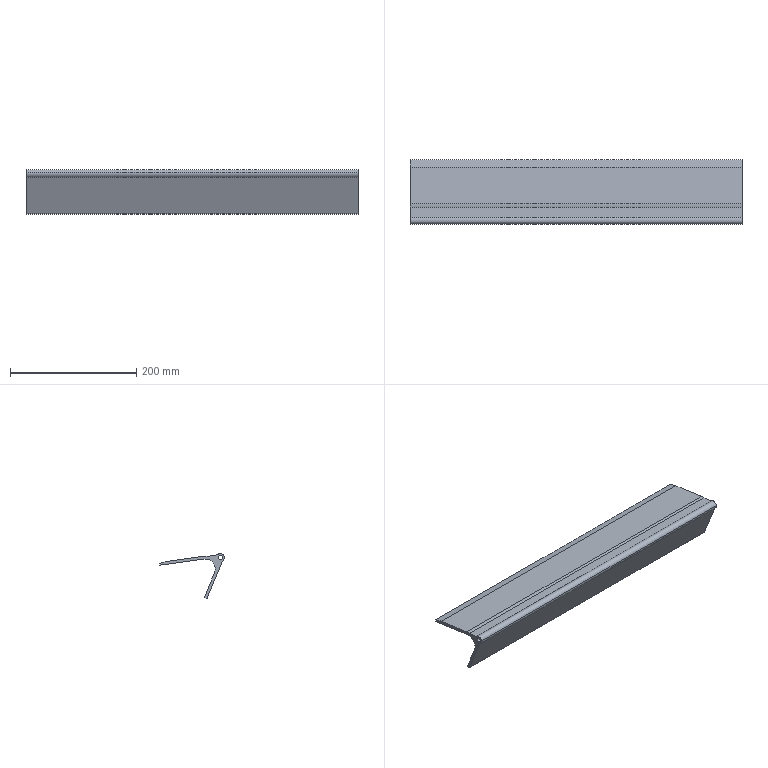Component | SolidWorks | DNR-71M20100BBEF2xx-A_501077-1 | 1 solid | 18 faces | box 525.45 x 102.87 x 71.23 mm | volume 480800 mm3 | plane 10 | cylinder 8 | commonest cylinder face diameters 12.7 x2 6.528 x2 31.496 x2 2.54 x1 40.64 x1
STEP:
#1=COLOUR_RGB('',0.7922,0.8196,0.9333);
#2=FILL_AREA_STYLE_COLOUR('',#1);
#3=FILL_AREA_STYLE('',(#2));
#4=SURFACE_STYLE_FILL_AREA(#3);
#5=SURFACE_SIDE_STYLE('',(#4));
#6=SURFACE_STYLE_USAGE(.BOTH.,#5);
#7=PRESENTATION_STYLE_ASSIGNMENT((#6));
#8=CARTESIAN_POINT('',(-10.343,-7.315,8.301));
#9=VERTEX_POINT('',#8);
#10=CARTESIAN_POINT('',(-10.343,-6.88,8.433));
#11=VERTEX_POINT('',#10);
#12=CARTESIAN_POINT('',(-10.343,-7.067,8.267));
#13=DIRECTION('',(-1.,-0.,0.));
#14=DIRECTION('',(0.,-0.9906,0.1369));
#15=AXIS2_PLACEMENT_3D('',#12,#13,#14);
#16=CIRCLE('',#15,0.25);
#17=EDGE_CURVE('',#9,#11,#16,.T.);
#18=ORIENTED_EDGE('',*,*,#17,.F.);
#19=CARTESIAN_POINT('',(10.343,-7.315,8.301));
#20=VERTEX_POINT('',#19);
#21=CARTESIAN_POINT('',(-11.051,-7.315,8.301));
#22=DIRECTION('',(1.,0.,-0.));
#23=VECTOR('',#22,39.37);
#24=LINE('',#21,#23);
#25=EDGE_CURVE('',#9,#20,#24,.T.);
#26=ORIENTED_EDGE('',*,*,#25,.T.);
#27=CARTESIAN_POINT('',(10.343,-6.88,8.433));
#28=VERTEX_POINT('',#27);
#29=CARTESIAN_POINT('',(10.343,-7.067,8.267));
#30=DIRECTION('',(1.,0.,-0.));
#31=DIRECTION('',(0.,-0.9906,0.1369));
#32=AXIS2_PLACEMENT_3D('',#29,#30,#31);
#33=CIRCLE('',#32,0.25);
#34=EDGE_CURVE('',#28,#20,#33,.T.);
#35=ORIENTED_EDGE('',*,*,#34,.F.);
#36=CARTESIAN_POINT('',(-11.051,-6.88,8.433));
#37=DIRECTION('',(-1.,-0.,0.));
#38=VECTOR('',#37,39.37);
#39=LINE('',#36,#38);
#40=EDGE_CURVE('',#28,#11,#39,.T.);
#41=ORIENTED_EDGE('',*,*,#40,.T.);
#42=EDGE_LOOP('',(#18,#26,#35,#41));
#43=FACE_OUTER_BOUND('',#42,.T.);
#44=CARTESIAN_POINT('',(-11.051,-7.067,8.267));
#45=DIRECTION('',(1.,0.,-0.));
#46=DIRECTION('',(0.,-0.9906,0.1369));
#47=AXIS2_PLACEMENT_3D('',#44,#45,#46);
#48=CYLINDRICAL_SURFACE('',#47,0.25);
#49=ADVANCED_FACE('',(#43),#48,.T.);
#50=CARTESIAN_POINT('',(-10.343,-7.194,8.285));
#51=VERTEX_POINT('',#50);
#52=CARTESIAN_POINT('',(-10.343,-6.94,8.25));
#53=VERTEX_POINT('',#52);
#54=CARTESIAN_POINT('',(-10.343,-7.067,8.267));
#55=DIRECTION('',(-1.,-0.,0.));
#56=DIRECTION('',(0.,-0.9906,0.1369));
#57=AXIS2_PLACEMENT_3D('',#54,#55,#56);
#58=CIRCLE('',#57,0.1285);
#59=EDGE_CURVE('',#51,#53,#58,.T.);
#60=ORIENTED_EDGE('',*,*,#59,.T.);
#61=CARTESIAN_POINT('',(10.343,-6.94,8.25));
#62=VERTEX_POINT('',#61);
#63=CARTESIAN_POINT('',(-11.891,-6.94,8.25));
#64=DIRECTION('',(1.,0.,-0.));
#65=VECTOR('',#64,39.37);
#66=LINE('',#63,#65);
#67=EDGE_CURVE('',#53,#62,#66,.T.);
#68=ORIENTED_EDGE('',*,*,#67,.T.);
#69=CARTESIAN_POINT('',(10.343,-7.194,8.285));
#70=VERTEX_POINT('',#69);
#71=CARTESIAN_POINT('',(10.343,-7.067,8.267));
#72=DIRECTION('',(1.,0.,-0.));
#73=DIRECTION('',(0.,-0.9906,0.1369));
#74=AXIS2_PLACEMENT_3D('',#71,#72,#73);
#75=CIRCLE('',#74,0.1285);
#76=EDGE_CURVE('',#62,#70,#75,.T.);
#77=ORIENTED_EDGE('',*,*,#76,.T.);
#78=CARTESIAN_POINT('',(-11.891,-7.194,8.285));
#79=DIRECTION('',(1.,0.,-0.));
#80=VECTOR('',#79,39.37);
#81=LINE('',#78,#80);
#82=EDGE_CURVE('',#51,#70,#81,.T.);
#83=ORIENTED_EDGE('',*,*,#82,.F.);
#84=EDGE_LOOP('',(#60,#68,#77,#83));
#85=FACE_OUTER_BOUND('',#84,.T.);
#86=CARTESIAN_POINT('',(-11.891,-7.067,8.267));
#87=DIRECTION('',(1.,0.,-0.));
#88=DIRECTION('',(0.,-0.9906,0.1369));
#89=AXIS2_PLACEMENT_3D('',#86,#87,#88);
#90=CYLINDRICAL_SURFACE('',#89,0.1285);
#91=ADVANCED_FACE('',(#85),#90,.F.);
#92=CARTESIAN_POINT('',(-10.343,-6.691,7.317));
#93=VERTEX_POINT('',#92);
#94=CARTESIAN_POINT('',(-10.343,-6.731,7.635));
#95=VERTEX_POINT('',#94);
#96=CARTESIAN_POINT('',(-10.343,-6.117,7.55));
#97=DIRECTION('',(-1.,-0.,0.));
#98=DIRECTION('',(0.,-0.9906,0.1369));
#99=AXIS2_PLACEMENT_3D('',#96,#97,#98);
#100=CIRCLE('',#99,0.62);
#101=EDGE_CURVE('',#93,#95,#100,.T.);
#102=ORIENTED_EDGE('',*,*,#101,.T.);
#103=CARTESIAN_POINT('',(10.343,-6.731,7.635));
#104=VERTEX_POINT('',#103);
#105=CARTESIAN_POINT('',(-10.343,-6.731,7.635));
#106=DIRECTION('',(1.,0.,-0.));
#107=VECTOR('',#106,39.37);
#108=LINE('',#105,#107);
#109=EDGE_CURVE('',#95,#104,#108,.T.);
#110=ORIENTED_EDGE('',*,*,#109,.T.);
#111=CARTESIAN_POINT('',(10.343,-6.691,7.317));
#112=VERTEX_POINT('',#111);
#113=CARTESIAN_POINT('',(10.343,-6.117,7.55));
#114=DIRECTION('',(-1.,-0.,0.));
#115=DIRECTION('',(0.,-0.9906,0.1369));
#116=AXIS2_PLACEMENT_3D('',#113,#114,#115);
#117=CIRCLE('',#116,0.62);
#118=EDGE_CURVE('',#112,#104,#117,.T.);
#119=ORIENTED_EDGE('',*,*,#118,.F.);
#120=CARTESIAN_POINT('',(-10.343,-6.691,7.317));
#121=DIRECTION('',(1.,0.,-0.));
#122=VECTOR('',#121,39.37);
#123=LINE('',#120,#122);
#124=EDGE_CURVE('',#93,#112,#123,.T.);
#125=ORIENTED_EDGE('',*,*,#124,.F.);
#126=EDGE_LOOP('',(#102,#110,#119,#125));
#127=FACE_OUTER_BOUND('',#126,.T.);
#128=CARTESIAN_POINT('',(-10.343,-6.117,7.55));
#129=DIRECTION('',(1.,0.,-0.));
#130=DIRECTION('',(0.,-0.9906,0.1369));
#131=AXIS2_PLACEMENT_3D('',#128,#129,#130);
#132=CYLINDRICAL_SURFACE('',#131,0.62);
#133=ADVANCED_FACE('',(#127),#132,.F.);
#134=CARTESIAN_POINT('',(10.343,-6.246,5.744));
#135=VERTEX_POINT('',#134);
#136=CARTESIAN_POINT('',(10.343,-6.181,5.716));
#137=VERTEX_POINT('',#136);
#138=CARTESIAN_POINT('',(10.343,-6.2,5.763));
#139=DIRECTION('',(1.,0.,-0.));
#140=DIRECTION('',(0.,-0.9906,0.1369));
#141=AXIS2_PLACEMENT_3D('',#138,#139,#140);
#142=CIRCLE('',#141,0.05);
#143=EDGE_CURVE('',#135,#137,#142,.T.);
#144=ORIENTED_EDGE('',*,*,#143,.F.);
#145=CARTESIAN_POINT('',(-10.343,-6.246,5.744));
#146=VERTEX_POINT('',#145);
#147=CARTESIAN_POINT('',(-10.343,-6.246,5.744));
#148=DIRECTION('',(1.,0.,-0.));
#149=VECTOR('',#148,39.37);
#150=LINE('',#147,#149);
#151=EDGE_CURVE('',#146,#135,#150,.T.);
#152=ORIENTED_EDGE('',*,*,#151,.F.);
#153=CARTESIAN_POINT('',(-10.343,-6.181,5.716));
#154=VERTEX_POINT('',#153);
#155=CARTESIAN_POINT('',(-10.343,-6.2,5.763));
#156=DIRECTION('',(1.,0.,-0.));
#157=DIRECTION('',(0.,-0.9906,0.1369));
#158=AXIS2_PLACEMENT_3D('',#155,#156,#157);
#159=CIRCLE('',#158,0.05);
#160=EDGE_CURVE('',#146,#154,#159,.T.);
#161=ORIENTED_EDGE('',*,*,#160,.T.);
#162=CARTESIAN_POINT('',(-10.343,-6.181,5.716));
#163=DIRECTION('',(1.,0.,-0.));
#164=VECTOR('',#163,39.37);
#165=LINE('',#162,#164);
#166=EDGE_CURVE('',#154,#137,#165,.T.);
#167=ORIENTED_EDGE('',*,*,#166,.T.);
#168=EDGE_LOOP('',(#144,#152,#161,#167));
#169=FACE_OUTER_BOUND('',#168,.T.);
#170=CARTESIAN_POINT('',(-10.343,-6.2,5.763));
#171=DIRECTION('',(1.,0.,-0.));
#172=DIRECTION('',(0.,-0.9906,0.1369));
#173=AXIS2_PLACEMENT_3D('',#170,#171,#172);
#174=CYLINDRICAL_SURFACE('',#173,0.05);
#175=ADVANCED_FACE('',(#169),#174,.T.);
#176=CARTESIAN_POINT('',(-10.343,-7.182,8.045));
#177=VERTEX_POINT('',#176);
#178=CARTESIAN_POINT('',(10.343,-7.182,8.045));
#179=VERTEX_POINT('',#178);
#180=CARTESIAN_POINT('',(-11.051,-7.182,8.045));
#181=DIRECTION('',(1.,0.,-0.));
#182=VECTOR('',#181,39.37);
#183=LINE('',#180,#182);
#184=EDGE_CURVE('',#177,#179,#183,.T.);
#185=ORIENTED_EDGE('',*,*,#184,.F.);
#186=CARTESIAN_POINT('',(-10.343,-6.858,7.249));
#187=DIRECTION('',(-0.,0.3767,-0.9263));
#188=VECTOR('',#187,39.37);
#189=LINE('',#186,#188);
#190=EDGE_CURVE('',#177,#146,#189,.T.);
#191=ORIENTED_EDGE('',*,*,#190,.T.);
#192=ORIENTED_EDGE('',*,*,#151,.T.);
#193=CARTESIAN_POINT('',(10.343,-6.858,7.249));
#194=DIRECTION('',(-0.,0.3767,-0.9263));
#195=VECTOR('',#194,39.37);
#196=LINE('',#193,#195);
#197=EDGE_CURVE('',#179,#135,#196,.T.);
#198=ORIENTED_EDGE('',*,*,#197,.F.);
#199=EDGE_LOOP('',(#185,#191,#192,#198));
#200=FACE_OUTER_BOUND('',#199,.T.);
#201=CARTESIAN_POINT('',(-10.343,-6.858,7.249));
#202=DIRECTION('',(0.,-0.9263,-0.3767));
#203=DIRECTION('',(-0.,0.3767,-0.9263));
#204=AXIS2_PLACEMENT_3D('',#201,#202,#203);
#205=PLANE('',#204);
#206=ADVANCED_FACE('',(#200),#205,.T.);
#207=CARTESIAN_POINT('',(-10.343,-6.227,8.343));
#208=VERTEX_POINT('',#207);
#209=CARTESIAN_POINT('',(10.343,-6.227,8.343));
#210=VERTEX_POINT('',#209);
#211=CARTESIAN_POINT('',(-11.891,-6.227,8.343));
#212=DIRECTION('',(1.,0.,-0.));
#213=VECTOR('',#212,39.37);
#214=LINE('',#211,#213);
#215=EDGE_CURVE('',#208,#210,#214,.T.);
#216=ORIENTED_EDGE('',*,*,#215,.T.);
#217=CARTESIAN_POINT('',(10.343,-6.007,8.343));
#218=VERTEX_POINT('',#217);
#219=CARTESIAN_POINT('',(10.343,-6.117,7.55));
#220=DIRECTION('',(1.,0.,-0.));
#221=DIRECTION('',(0.,-0.9906,0.1369));
#222=AXIS2_PLACEMENT_3D('',#219,#220,#221);
#223=CIRCLE('',#222,0.8);
#224=EDGE_CURVE('',#218,#210,#223,.T.);
#225=ORIENTED_EDGE('',*,*,#224,.F.);
#226=CARTESIAN_POINT('',(-10.343,-6.007,8.343));
#227=VERTEX_POINT('',#226);
#228=CARTESIAN_POINT('',(-10.343,-6.007,8.343));
#229=DIRECTION('',(1.,0.,-0.));
#230=VECTOR('',#229,39.37);
#231=LINE('',#228,#230);
#232=EDGE_CURVE('',#227,#218,#231,.T.);
#233=ORIENTED_EDGE('',*,*,#232,.F.);
#234=CARTESIAN_POINT('',(-10.343,-6.117,7.55));
#235=DIRECTION('',(1.,0.,-0.));
#236=DIRECTION('',(0.,-0.9906,0.1369));
#237=AXIS2_PLACEMENT_3D('',#234,#235,#236);
#238=CIRCLE('',#237,0.8);
#239=EDGE_CURVE('',#227,#208,#238,.T.);
#240=ORIENTED_EDGE('',*,*,#239,.T.);
#241=EDGE_LOOP('',(#216,#225,#233,#240));
#242=FACE_OUTER_BOUND('',#241,.T.);
#243=CARTESIAN_POINT('',(-10.343,-6.117,7.55));
#244=DIRECTION('',(1.,0.,-0.));
#245=DIRECTION('',(0.,-0.9906,0.1369));
#246=AXIS2_PLACEMENT_3D('',#243,#244,#245);
#247=CYLINDRICAL_SURFACE('',#246,0.8);
#248=ADVANCED_FACE('',(#242),#247,.T.);
#249=CARTESIAN_POINT('',(10.343,-3.754,8.031));
#250=VERTEX_POINT('',#249);
#251=CARTESIAN_POINT('',(10.343,-6.007,8.343));
#252=DIRECTION('',(0.,-0.9906,0.1369));
#253=VECTOR('',#252,39.37);
#254=LINE('',#251,#253);
#255=EDGE_CURVE('',#250,#218,#254,.T.);
#256=ORIENTED_EDGE('',*,*,#255,.F.);
#257=CARTESIAN_POINT('',(-10.343,-3.754,8.031));
#258=VERTEX_POINT('',#257);
#259=CARTESIAN_POINT('',(-10.343,-3.754,8.031));
#260=DIRECTION('',(1.,0.,-0.));
#261=VECTOR('',#260,39.37);
#262=LINE('',#259,#261);
#263=EDGE_CURVE('',#258,#250,#262,.T.);
#264=ORIENTED_EDGE('',*,*,#263,.F.);
#265=CARTESIAN_POINT('',(-10.343,-6.007,8.343));
#266=DIRECTION('',(0.,-0.9906,0.1369));
#267=VECTOR('',#266,39.37);
#268=LINE('',#265,#267);
#269=EDGE_CURVE('',#258,#227,#268,.T.);
#270=ORIENTED_EDGE('',*,*,#269,.T.);
#271=ORIENTED_EDGE('',*,*,#232,.T.);
#272=EDGE_LOOP('',(#256,#264,#270,#271));
#273=FACE_OUTER_BOUND('',#272,.T.);
#274=CARTESIAN_POINT('',(-10.343,-6.007,8.343));
#275=DIRECTION('',(0.,0.1369,0.9906));
#276=DIRECTION('',(0.,-0.9906,0.1369));
#277=AXIS2_PLACEMENT_3D('',#274,#275,#276);
#278=PLANE('',#277);
#279=ADVANCED_FACE('',(#273),#278,.T.);
#280=CARTESIAN_POINT('',(10.343,-3.267,7.901));
#281=VERTEX_POINT('',#280);
#282=CARTESIAN_POINT('',(10.343,-3.267,7.901));
#283=DIRECTION('',(0.,-0.9662,0.2579));
#284=VECTOR('',#283,39.37);
#285=LINE('',#282,#284);
#286=EDGE_CURVE('',#281,#250,#285,.T.);
#287=ORIENTED_EDGE('',*,*,#286,.F.);
#288=CARTESIAN_POINT('',(-10.343,-3.267,7.901));
#289=VERTEX_POINT('',#288);
#290=CARTESIAN_POINT('',(-10.343,-3.267,7.901));
#291=DIRECTION('',(1.,0.,-0.));
#292=VECTOR('',#291,39.37);
#293=LINE('',#290,#292);
#294=EDGE_CURVE('',#289,#281,#293,.T.);
#295=ORIENTED_EDGE('',*,*,#294,.F.);
#296=CARTESIAN_POINT('',(-10.343,-3.267,7.901));
#297=DIRECTION('',(0.,-0.9662,0.2579));
#298=VECTOR('',#297,39.37);
#299=LINE('',#296,#298);
#300=EDGE_CURVE('',#289,#258,#299,.T.);
#301=ORIENTED_EDGE('',*,*,#300,.T.);
#302=ORIENTED_EDGE('',*,*,#263,.T.);
#303=EDGE_LOOP('',(#287,#295,#301,#302));
#304=FACE_OUTER_BOUND('',#303,.T.);
#305=CARTESIAN_POINT('',(-10.343,-3.267,7.901));
#306=DIRECTION('',(0.,0.2579,0.9662));
#307=DIRECTION('',(0.,-0.9662,0.2579));
#308=AXIS2_PLACEMENT_3D('',#305,#306,#307);
#309=PLANE('',#308);
#310=ADVANCED_FACE('',(#304),#309,.T.);
#311=CARTESIAN_POINT('',(10.343,-3.283,7.784));
#312=VERTEX_POINT('',#311);
#313=CARTESIAN_POINT('',(10.343,-3.283,7.784));
#314=DIRECTION('',(0.,0.1369,0.9906));
#315=VECTOR('',#314,39.37);
#316=LINE('',#313,#315);
#317=EDGE_CURVE('',#312,#281,#316,.T.);
#318=ORIENTED_EDGE('',*,*,#317,.F.);
#319=CARTESIAN_POINT('',(-10.343,-3.283,7.784));
#320=VERTEX_POINT('',#319);
#321=CARTESIAN_POINT('',(-10.343,-3.283,7.784));
#322=DIRECTION('',(1.,0.,-0.));
#323=VECTOR('',#322,39.37);
#324=LINE('',#321,#323);
#325=EDGE_CURVE('',#320,#312,#324,.T.);
#326=ORIENTED_EDGE('',*,*,#325,.F.);
#327=CARTESIAN_POINT('',(-10.343,-3.283,7.784));
#328=DIRECTION('',(0.,0.1369,0.9906));
#329=VECTOR('',#328,39.37);
#330=LINE('',#327,#329);
#331=EDGE_CURVE('',#320,#289,#330,.T.);
#332=ORIENTED_EDGE('',*,*,#331,.T.);
#333=ORIENTED_EDGE('',*,*,#294,.T.);
#334=EDGE_LOOP('',(#318,#326,#332,#333));
#335=FACE_OUTER_BOUND('',#334,.T.);
#336=CARTESIAN_POINT('',(-10.343,-3.283,7.784));
#337=DIRECTION('',(-0.,0.9906,-0.1369));
#338=DIRECTION('',(1.,0.,-0.));
#339=AXIS2_PLACEMENT_3D('',#336,#337,#338);
#340=PLANE('',#339);
#341=ADVANCED_FACE('',(#335),#340,.T.);
#342=CARTESIAN_POINT('',(10.343,-6.032,8.164));
#343=VERTEX_POINT('',#342);
#344=CARTESIAN_POINT('',(10.343,-6.032,8.164));
#345=DIRECTION('',(-0.,0.9906,-0.1369));
#346=VECTOR('',#345,39.37);
#347=LINE('',#344,#346);
#348=EDGE_CURVE('',#343,#312,#347,.T.);
#349=ORIENTED_EDGE('',*,*,#348,.F.);
#350=CARTESIAN_POINT('',(-10.343,-6.032,8.164));
#351=VERTEX_POINT('',#350);
#352=CARTESIAN_POINT('',(-10.343,-6.032,8.164));
#353=DIRECTION('',(1.,0.,-0.));
#354=VECTOR('',#353,39.37);
#355=LINE('',#352,#354);
#356=EDGE_CURVE('',#351,#343,#355,.T.);
#357=ORIENTED_EDGE('',*,*,#356,.F.);
#358=CARTESIAN_POINT('',(-10.343,-6.032,8.164));
#359=DIRECTION('',(-0.,0.9906,-0.1369));
#360=VECTOR('',#359,39.37);
#361=LINE('',#358,#360);
#362=EDGE_CURVE('',#351,#320,#361,.T.);
#363=ORIENTED_EDGE('',*,*,#362,.T.);
#364=ORIENTED_EDGE('',*,*,#325,.T.);
#365=EDGE_LOOP('',(#349,#357,#363,#364));
#366=FACE_OUTER_BOUND('',#365,.T.);
#367=CARTESIAN_POINT('',(-10.343,-6.032,8.164));
#368=DIRECTION('',(-0.,-0.1369,-0.9906));
#369=DIRECTION('',(-0.,0.9906,-0.1369));
#370=AXIS2_PLACEMENT_3D('',#367,#368,#369);
#371=PLANE('',#370);
#372=ADVANCED_FACE('',(#366),#371,.T.);
#373=ORIENTED_EDGE('',*,*,#109,.F.);
#374=CARTESIAN_POINT('',(-10.343,-6.117,7.55));
#375=DIRECTION('',(-1.,-0.,0.));
#376=DIRECTION('',(0.,-0.9906,0.1369));
#377=AXIS2_PLACEMENT_3D('',#374,#375,#376);
#378=CIRCLE('',#377,0.62);
#379=EDGE_CURVE('',#95,#351,#378,.T.);
#380=ORIENTED_EDGE('',*,*,#379,.T.);
#381=ORIENTED_EDGE('',*,*,#356,.T.);
#382=CARTESIAN_POINT('',(10.343,-6.117,7.55));
#383=DIRECTION('',(-1.,-0.,0.));
#384=DIRECTION('',(0.,-0.9906,0.1369));
#385=AXIS2_PLACEMENT_3D('',#382,#383,#384);
#386=CIRCLE('',#385,0.62);
#387=EDGE_CURVE('',#104,#343,#386,.T.);
#388=ORIENTED_EDGE('',*,*,#387,.F.);
#389=EDGE_LOOP('',(#373,#380,#381,#388));
#390=FACE_OUTER_BOUND('',#389,.T.);
#391=CARTESIAN_POINT('',(-10.343,-6.117,7.55));
#392=DIRECTION('',(1.,0.,-0.));
#393=DIRECTION('',(0.,-0.9906,0.1369));
#394=AXIS2_PLACEMENT_3D('',#391,#392,#393);
#395=CYLINDRICAL_SURFACE('',#394,0.62);
#396=ADVANCED_FACE('',(#390),#395,.F.);
#397=CARTESIAN_POINT('',(10.343,-6.06,5.765));
#398=VERTEX_POINT('',#397);
#399=CARTESIAN_POINT('',(10.343,-6.691,7.317));
#400=DIRECTION('',(0.,-0.3767,0.9263));
#401=VECTOR('',#400,39.37);
#402=LINE('',#399,#401);
#403=EDGE_CURVE('',#398,#112,#402,.T.);
#404=ORIENTED_EDGE('',*,*,#403,.F.);
#405=CARTESIAN_POINT('',(-10.343,-6.06,5.765));
#406=VERTEX_POINT('',#405);
#407=CARTESIAN_POINT('',(-10.343,-6.06,5.765));
#408=DIRECTION('',(1.,0.,-0.));
#409=VECTOR('',#408,39.37);
#410=LINE('',#407,#409);
#411=EDGE_CURVE('',#406,#398,#410,.T.);
#412=ORIENTED_EDGE('',*,*,#411,.F.);
#413=CARTESIAN_POINT('',(-10.343,-6.691,7.317));
#414=DIRECTION('',(0.,-0.3767,0.9263));
#415=VECTOR('',#414,39.37);
#416=LINE('',#413,#415);
#417=EDGE_CURVE('',#406,#93,#416,.T.);
#418=ORIENTED_EDGE('',*,*,#417,.T.);
#419=ORIENTED_EDGE('',*,*,#124,.T.);
#420=EDGE_LOOP('',(#404,#412,#418,#419));
#421=FACE_OUTER_BOUND('',#420,.T.);
#422=CARTESIAN_POINT('',(-10.343,-6.691,7.317));
#423=DIRECTION('',(-0.,0.9263,0.3767));
#424=DIRECTION('',(0.,-0.3767,0.9263));
#425=AXIS2_PLACEMENT_3D('',#422,#423,#424);
#426=PLANE('',#425);
#427=ADVANCED_FACE('',(#421),#426,.T.);
#428=CARTESIAN_POINT('',(10.343,-6.06,5.765));
#429=DIRECTION('',(-0.,0.9263,0.3767));
#430=VECTOR('',#429,39.37);
#431=LINE('',#428,#430);
#432=EDGE_CURVE('',#137,#398,#431,.T.);
#433=ORIENTED_EDGE('',*,*,#432,.F.);
#434=ORIENTED_EDGE('',*,*,#166,.F.);
#435=CARTESIAN_POINT('',(-10.343,-6.06,5.765));
#436=DIRECTION('',(-0.,0.9263,0.3767));
#437=VECTOR('',#436,39.37);
#438=LINE('',#435,#437);
#439=EDGE_CURVE('',#154,#406,#438,.T.);
#440=ORIENTED_EDGE('',*,*,#439,.T.);
#441=ORIENTED_EDGE('',*,*,#411,.T.);
#442=EDGE_LOOP('',(#433,#434,#440,#441));
#443=FACE_OUTER_BOUND('',#442,.T.);
#444=CARTESIAN_POINT('',(-10.343,-6.06,5.765));
#445=DIRECTION('',(-0.,0.3767,-0.9263));
#446=DIRECTION('',(-0.,0.9263,0.3767));
#447=AXIS2_PLACEMENT_3D('',#444,#445,#446);
#448=PLANE('',#447);
#449=ADVANCED_FACE('',(#443),#448,.T.);
#450=ORIENTED_EDGE('',*,*,#190,.F.);
#451=CARTESIAN_POINT('',(-10.343,-7.067,8.267));
#452=DIRECTION('',(-1.,-0.,0.));
#453=DIRECTION('',(0.,-0.9906,0.1369));
#454=AXIS2_PLACEMENT_3D('',#451,#452,#453);
#455=CIRCLE('',#454,0.25);
#456=EDGE_CURVE('',#177,#9,#455,.T.);
#457=ORIENTED_EDGE('',*,*,#456,.T.);
#458=ORIENTED_EDGE('',*,*,#17,.T.);
#459=CARTESIAN_POINT('',(-10.343,-6.227,8.343));
#460=DIRECTION('',(-0.,0.9906,-0.1369));
#461=VECTOR('',#460,39.37);
#462=LINE('',#459,#461);
#463=EDGE_CURVE('',#11,#208,#462,.T.);
#464=ORIENTED_EDGE('',*,*,#463,.T.);
#465=ORIENTED_EDGE('',*,*,#239,.F.);
#466=ORIENTED_EDGE('',*,*,#269,.F.);
#467=ORIENTED_EDGE('',*,*,#300,.F.);
#468=ORIENTED_EDGE('',*,*,#331,.F.);
#469=ORIENTED_EDGE('',*,*,#362,.F.);
#470=ORIENTED_EDGE('',*,*,#379,.F.);
#471=ORIENTED_EDGE('',*,*,#101,.F.);
#472=ORIENTED_EDGE('',*,*,#417,.F.);
#473=ORIENTED_EDGE('',*,*,#439,.F.);
#474=ORIENTED_EDGE('',*,*,#160,.F.);
#475=EDGE_LOOP('',(#450,#457,#458,#464,#465,#466,#467,#468,#469,#470,#471,#472,#473,#474));
#476=FACE_OUTER_BOUND('',#475,.T.);
#477=ORIENTED_EDGE('',*,*,#59,.F.);
#478=CARTESIAN_POINT('',(-10.343,-7.067,8.267));
#479=DIRECTION('',(-1.,-0.,0.));
#480=DIRECTION('',(0.,-0.9906,0.1369));
#481=AXIS2_PLACEMENT_3D('',#478,#479,#480);
#482=CIRCLE('',#481,0.1285);
#483=EDGE_CURVE('',#53,#51,#482,.T.);
#484=ORIENTED_EDGE('',*,*,#483,.F.);
#485=EDGE_LOOP('',(#477,#484));
#486=FACE_BOUND('',#485,.T.);
#487=CARTESIAN_POINT('',(-10.343,-6.2,5.763));
#488=DIRECTION('',(1.,0.,-0.));
#489=DIRECTION('',(0.,-0.9906,0.1369));
#490=AXIS2_PLACEMENT_3D('',#487,#488,#489);
#491=PLANE('',#490);
#492=ADVANCED_FACE('',(#476,#486),#491,.F.);
#493=ORIENTED_EDGE('',*,*,#34,.T.);
#494=CARTESIAN_POINT('',(10.343,-7.067,8.267));
#495=DIRECTION('',(1.,0.,-0.));
#496=DIRECTION('',(0.,-0.9906,0.1369));
#497=AXIS2_PLACEMENT_3D('',#494,#495,#496);
#498=CIRCLE('',#497,0.25);
#499=EDGE_CURVE('',#20,#179,#498,.T.);
#500=ORIENTED_EDGE('',*,*,#499,.T.);
#501=ORIENTED_EDGE('',*,*,#197,.T.);
#502=ORIENTED_EDGE('',*,*,#143,.T.);
#503=ORIENTED_EDGE('',*,*,#432,.T.);
#504=ORIENTED_EDGE('',*,*,#403,.T.);
#505=ORIENTED_EDGE('',*,*,#118,.T.);
#506=ORIENTED_EDGE('',*,*,#387,.T.);
#507=ORIENTED_EDGE('',*,*,#348,.T.);
#508=ORIENTED_EDGE('',*,*,#317,.T.);
#509=ORIENTED_EDGE('',*,*,#286,.T.);
#510=ORIENTED_EDGE('',*,*,#255,.T.);
#511=ORIENTED_EDGE('',*,*,#224,.T.);
#512=CARTESIAN_POINT('',(10.343,-6.227,8.343));
#513=DIRECTION('',(0.,-0.9906,0.1369));
#514=VECTOR('',#513,39.37);
#515=LINE('',#512,#514);
#516=EDGE_CURVE('',#210,#28,#515,.T.);
#517=ORIENTED_EDGE('',*,*,#516,.T.);
#518=EDGE_LOOP('',(#493,#500,#501,#502,#503,#504,#505,#506,#507,#508,#509,#510,#511,#517));
#519=FACE_OUTER_BOUND('',#518,.T.);
#520=CARTESIAN_POINT('',(10.343,-7.067,8.267));
#521=DIRECTION('',(1.,0.,-0.));
#522=DIRECTION('',(0.,-0.9906,0.1369));
#523=AXIS2_PLACEMENT_3D('',#520,#521,#522);
#524=CIRCLE('',#523,0.1285);
#525=EDGE_CURVE('',#70,#62,#524,.T.);
#526=ORIENTED_EDGE('',*,*,#525,.F.);
#527=ORIENTED_EDGE('',*,*,#76,.F.);
#528=EDGE_LOOP('',(#526,#527));
#529=FACE_BOUND('',#528,.T.);
#530=CARTESIAN_POINT('',(10.343,-6.2,5.763));
#531=DIRECTION('',(1.,0.,-0.));
#532=DIRECTION('',(0.,-0.9906,0.1369));
#533=AXIS2_PLACEMENT_3D('',#530,#531,#532);
#534=PLANE('',#533);
#535=ADVANCED_FACE('',(#519,#529),#534,.T.);
#536=ORIENTED_EDGE('',*,*,#40,.F.);
#537=ORIENTED_EDGE('',*,*,#516,.F.);
#538=ORIENTED_EDGE('',*,*,#215,.F.);
#539=ORIENTED_EDGE('',*,*,#463,.F.);
#540=EDGE_LOOP('',(#536,#537,#538,#539));
#541=FACE_OUTER_BOUND('',#540,.T.);
#542=CARTESIAN_POINT('',(-11.891,-6.227,8.343));
#543=DIRECTION('',(0.,0.1369,0.9906));
#544=DIRECTION('',(0.,-0.9906,0.1369));
#545=AXIS2_PLACEMENT_3D('',#542,#543,#544);
#546=PLANE('',#545);
#547=ADVANCED_FACE('',(#541),#546,.T.);
#548=ORIENTED_EDGE('',*,*,#67,.F.);
#549=ORIENTED_EDGE('',*,*,#483,.T.);
#550=ORIENTED_EDGE('',*,*,#82,.T.);
#551=ORIENTED_EDGE('',*,*,#525,.T.);
#552=EDGE_LOOP('',(#548,#549,#550,#551));
#553=FACE_OUTER_BOUND('',#552,.T.);
#554=CARTESIAN_POINT('',(-11.891,-7.067,8.267));
#555=DIRECTION('',(1.,0.,-0.));
#556=DIRECTION('',(0.,-0.9906,0.1369));
#557=AXIS2_PLACEMENT_3D('',#554,#555,#556);
#558=CYLINDRICAL_SURFACE('',#557,0.1285);
#559=ADVANCED_FACE('',(#553),#558,.F.);
#560=ORIENTED_EDGE('',*,*,#25,.F.);
#561=ORIENTED_EDGE('',*,*,#456,.F.);
#562=ORIENTED_EDGE('',*,*,#184,.T.);
#563=ORIENTED_EDGE('',*,*,#499,.F.);
#564=EDGE_LOOP('',(#560,#561,#562,#563));
#565=FACE_OUTER_BOUND('',#564,.T.);
#566=CARTESIAN_POINT('',(-11.051,-7.067,8.267));
#567=DIRECTION('',(1.,0.,-0.));
#568=DIRECTION('',(0.,-0.9906,0.1369));
#569=AXIS2_PLACEMENT_3D('',#566,#567,#568);
#570=CYLINDRICAL_SURFACE('',#569,0.25);
#571=ADVANCED_FACE('',(#565),#570,.T.);
#572=CLOSED_SHELL('',(#49,#91,#133,#175,#206,#248,#279,#310,#341,#372,#396,#427,#449,#492,#535,#547,#559,#571));
#573=MANIFOLD_SOLID_BREP('',#572);
#574=STYLED_ITEM('',(#7),#573);
#575=(LENGTH_UNIT()NAMED_UNIT(*)SI_UNIT($,.METRE.));
#576=LENGTH_MEASURE_WITH_UNIT(LENGTH_MEASURE(0.0254),#575);
#577=DIMENSIONAL_EXPONENTS(1.,0.,0.,0.,0.,0.,0.);
#578=(CONVERSION_BASED_UNIT('',#576)LENGTH_UNIT()NAMED_UNIT(#577));
#579=UNCERTAINTY_MEASURE_WITH_UNIT(LENGTH_MEASURE(0.00001),#578,'','');
#580=(NAMED_UNIT(*)PLANE_ANGLE_UNIT()SI_UNIT($,.RADIAN.));
#581=(NAMED_UNIT(*)SI_UNIT($,.STERADIAN.)SOLID_ANGLE_UNIT());
#582=(GEOMETRIC_REPRESENTATION_CONTEXT(3)GLOBAL_UNCERTAINTY_ASSIGNED_CONTEXT((#579))GLOBAL_UNIT_ASSIGNED_CONTEXT((#578,#580,#581))REPRESENTATION_CONTEXT('',''));
#583=MECHANICAL_DESIGN_GEOMETRIC_PRESENTATION_REPRESENTATION('',(#574),#582);
#584=PRESENTATION_LAYER_ASSIGNMENT('','',(#574));
#585=CARTESIAN_POINT('',(0.,0.,0.));
#586=DIRECTION('',(0.,0.,1.));
#587=DIRECTION('',(1.,0.,0.));
#588=AXIS2_PLACEMENT_3D('',#585,#586,#587);
#589=(LENGTH_UNIT()NAMED_UNIT(*)SI_UNIT($,.METRE.));
#590=LENGTH_MEASURE_WITH_UNIT(LENGTH_MEASURE(0.0254),#589);
#591=DIMENSIONAL_EXPONENTS(1.,0.,0.,0.,0.,0.,0.);
#592=(CONVERSION_BASED_UNIT('',#590)LENGTH_UNIT()NAMED_UNIT(#591));
#593=UNCERTAINTY_MEASURE_WITH_UNIT(LENGTH_MEASURE(0.00001),#592,'','');
#594=(NAMED_UNIT(*)PLANE_ANGLE_UNIT()SI_UNIT($,.RADIAN.));
#595=(NAMED_UNIT(*)SI_UNIT($,.STERADIAN.)SOLID_ANGLE_UNIT());
#596=(GEOMETRIC_REPRESENTATION_CONTEXT(3)GLOBAL_UNCERTAINTY_ASSIGNED_CONTEXT((#593))GLOBAL_UNIT_ASSIGNED_CONTEXT((#592,#594,#595))REPRESENTATION_CONTEXT('',''));
#597=ADVANCED_BREP_SHAPE_REPRESENTATION('',(#573,#588),#596);